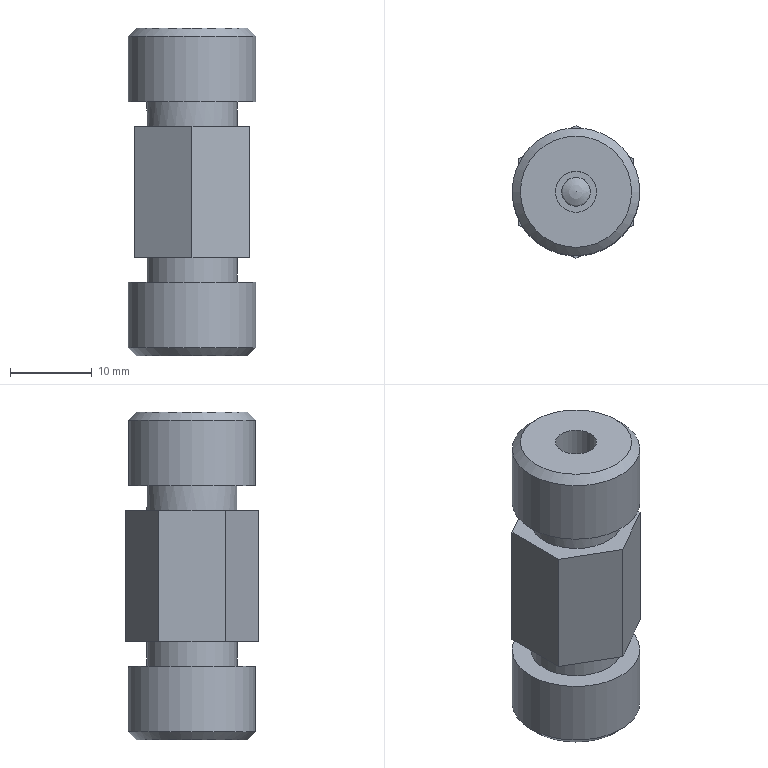Assembly | NX | mm | 5 component files | 5 solids | 63 faces | box 15.57 x 16.17 x 40 mm | volume 5923 mm3 | plane 35 | cylinder 13 | cone 8 | spline 5 | sphere 2 | commonest cylinder face diameters 6 x3 15.568 x2 11 x2 7.785 x2 5 x1 3.5 x1 6.5 x1 3 x1
Bill of materials:
unnamed part 1 | 1 |  | Open helical coil of round-section wire with constant coil diameter and roughly ten turns. The end turns look flattened into planar end faces. Its shape is consistent with a helical compression spring.
unnamed part 2 | 1 |  | Plain solid sphere with no visible holes, flats or other features.
unnamed part 3 | 1 |  | Axially symmetric part with a straight through-bore. It has a hexagonal middle section, a narrow necked groove on each side of the hex, and a cylindrical collar at each end with chamfered outer edges.
unnamed part 4 | 1 |  | Short cylindrical sleeve with chamfered ends and a central through-bore. Each end has a larger counterbore above an internal ledge. Two diametrically opposite axial slots run along the outer wall.
unnamed part 5 | 1 |  | Solid straight cylinder with a concave, roughly hemispherical or dished blind recess in one end face, leaving a thin flat annular rim.
Mates:
1. fix | DXF_01_valve_body 1 component
2. touch align | ball_6 1 face | DXF_02_spring_bracket 1 face
3. touch align | DXF_02_spring_bracket 1 face | DXF_01_valve_body 1 face
4. touch align | DXF_04_adjusting_screw 1 face | DXF_01_valve_body 1 face
5. touch align | DXF_03_compression_spring 1 datumaxis | DXF_04_adjusting_screw 1 face
6. touch align | DXF_03_compression_spring 1 face | DXF_04_adjusting_screw 1 face
7. touch align | DXF_02_spring_bracket 1 face | DXF_03_compression_spring 1 face
8. touch align | ball_6 1 face | DXF_01_valve_body 1 face